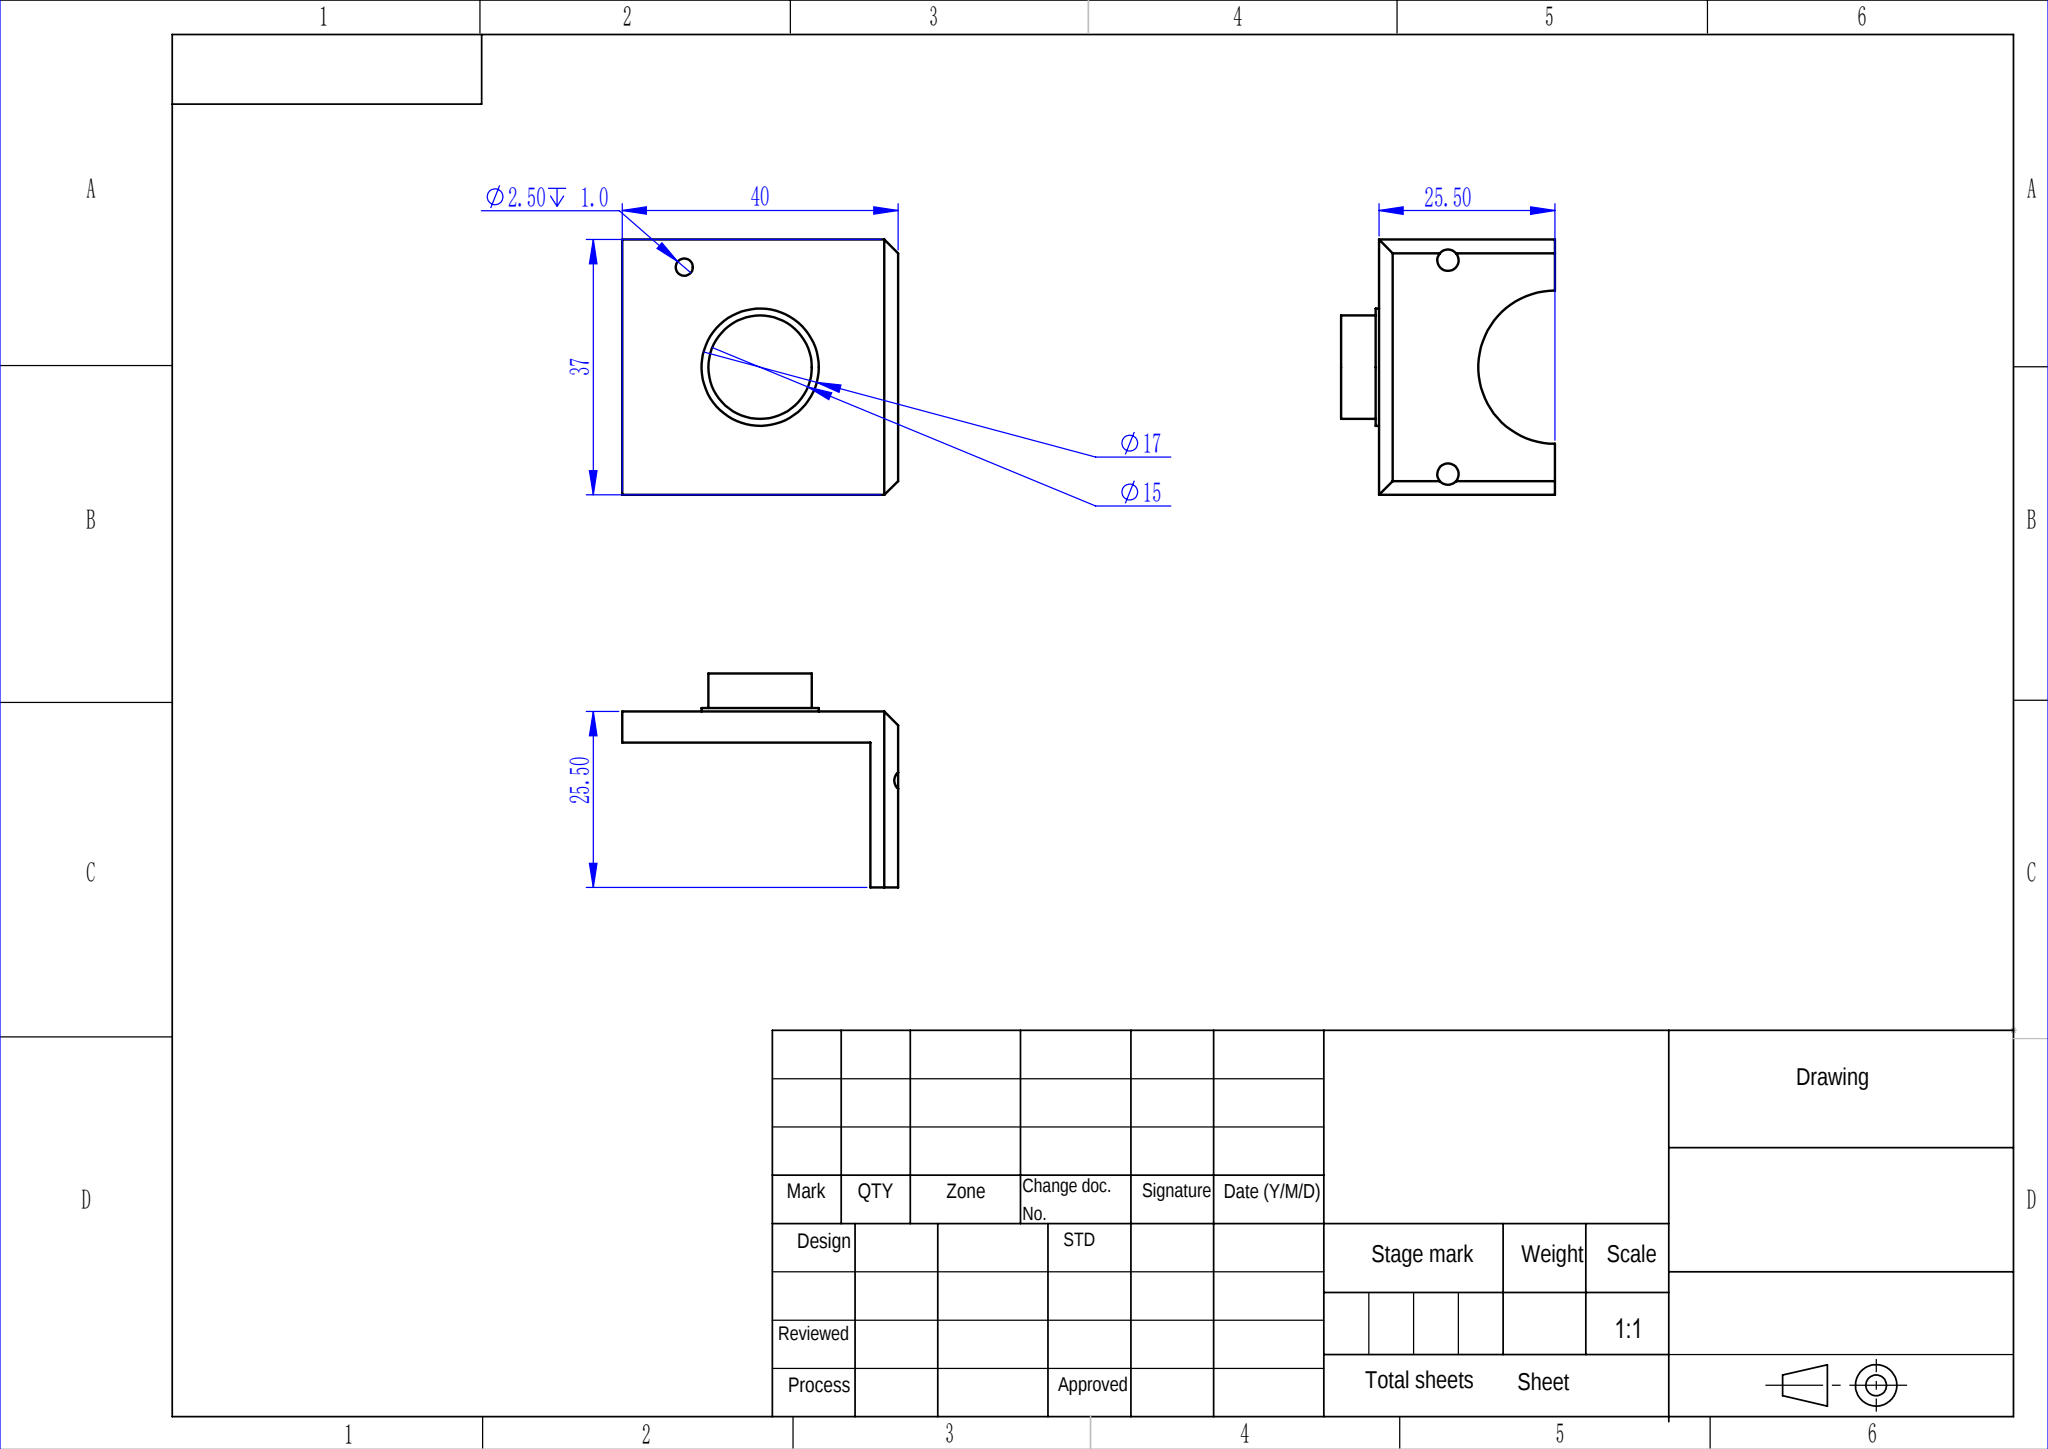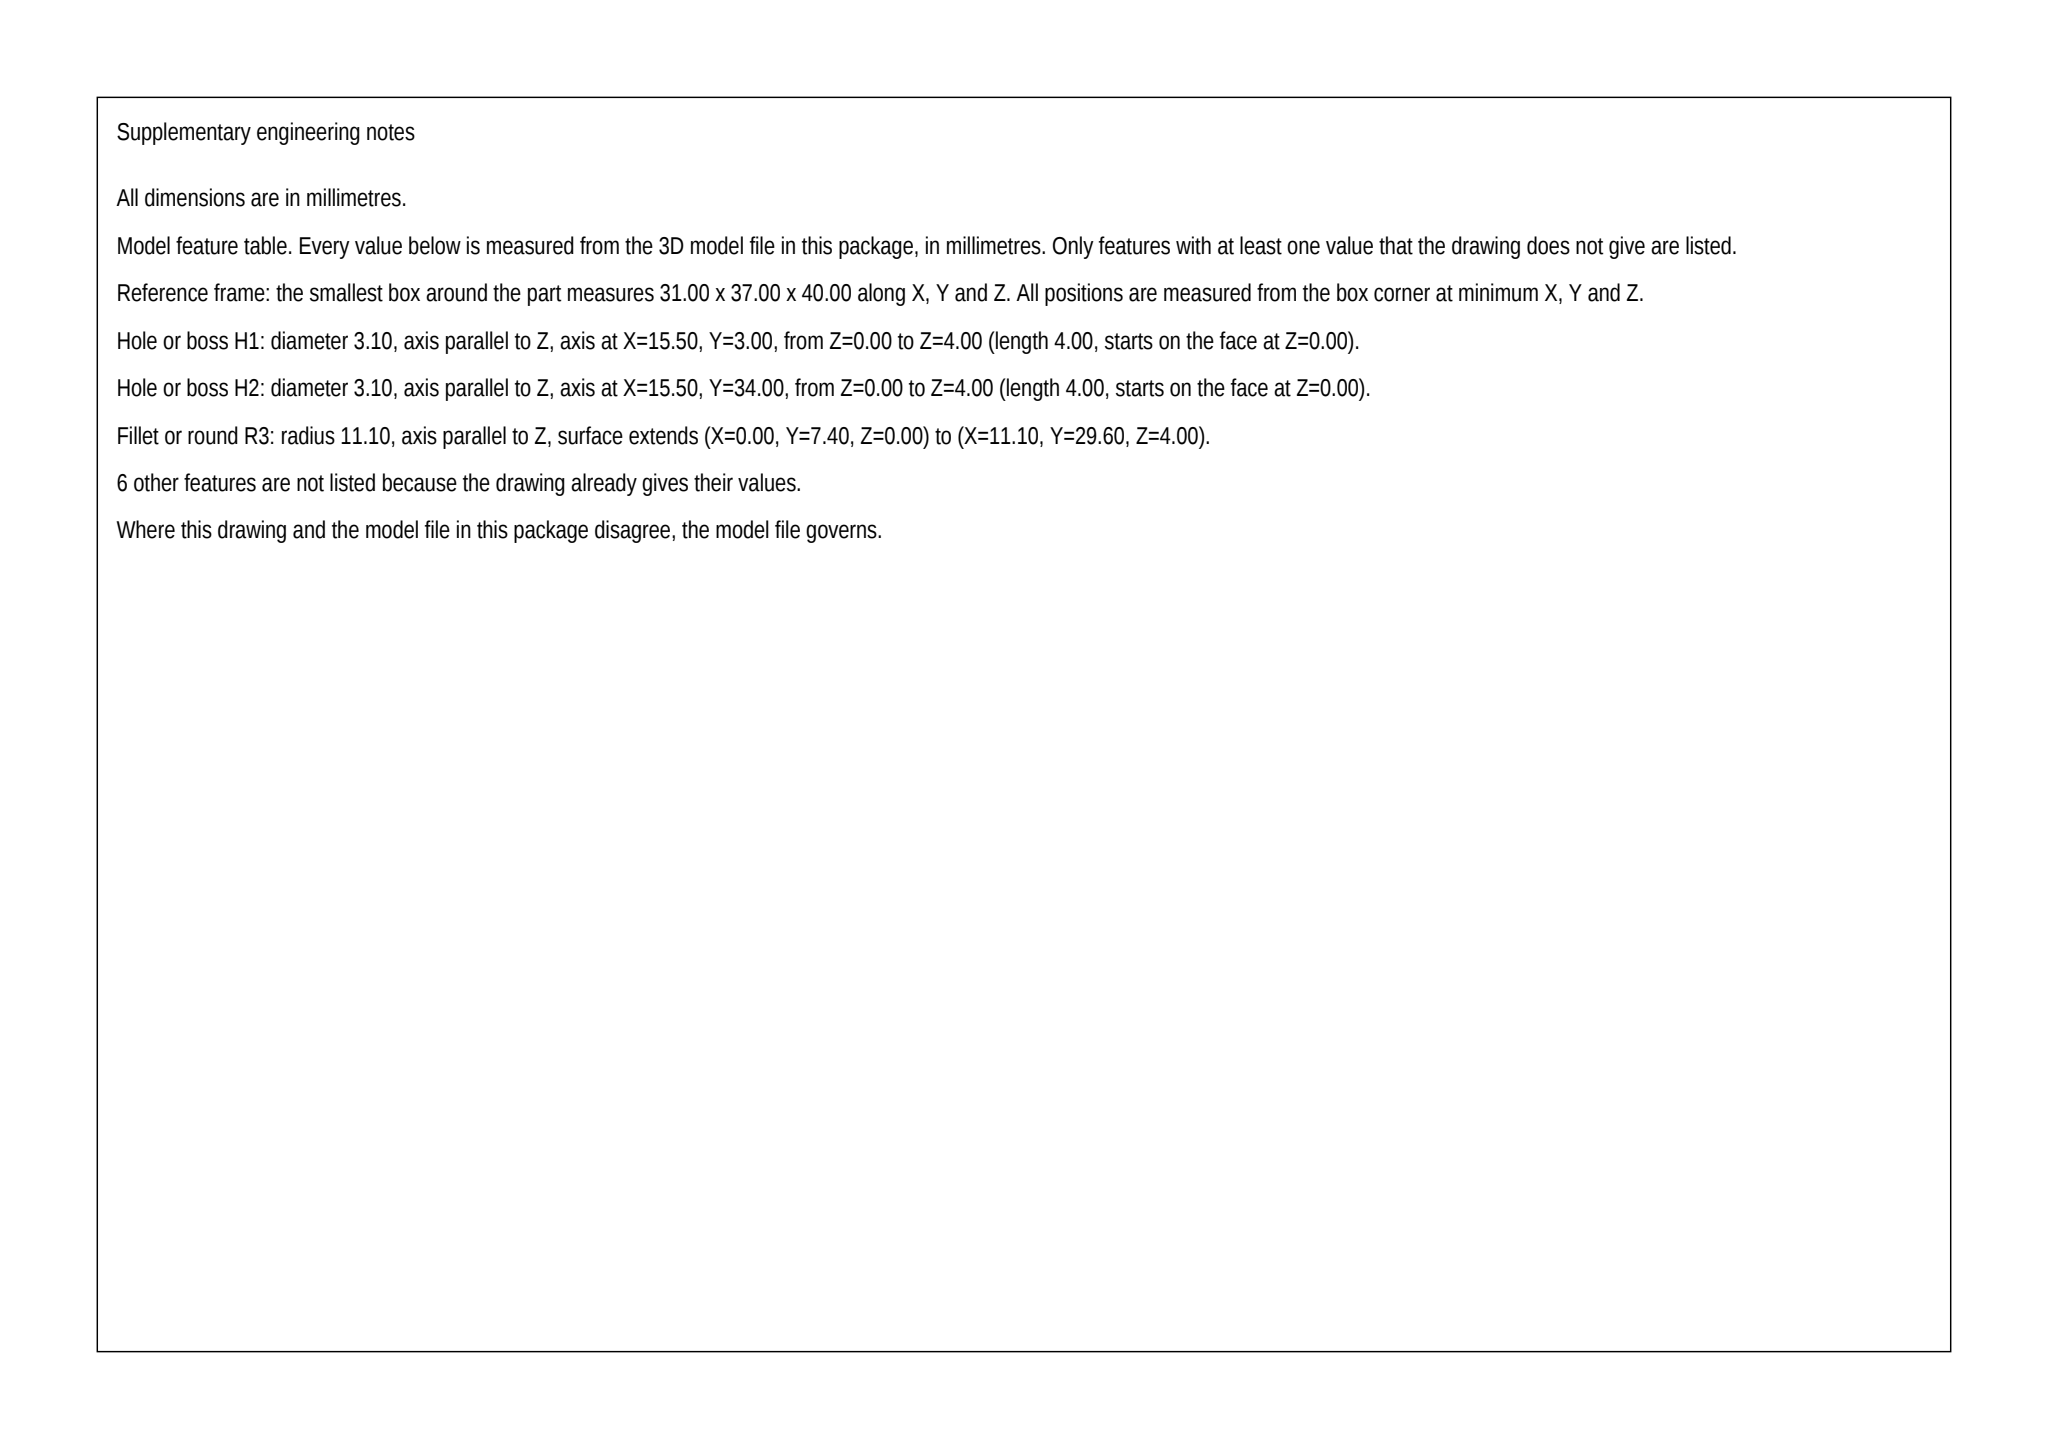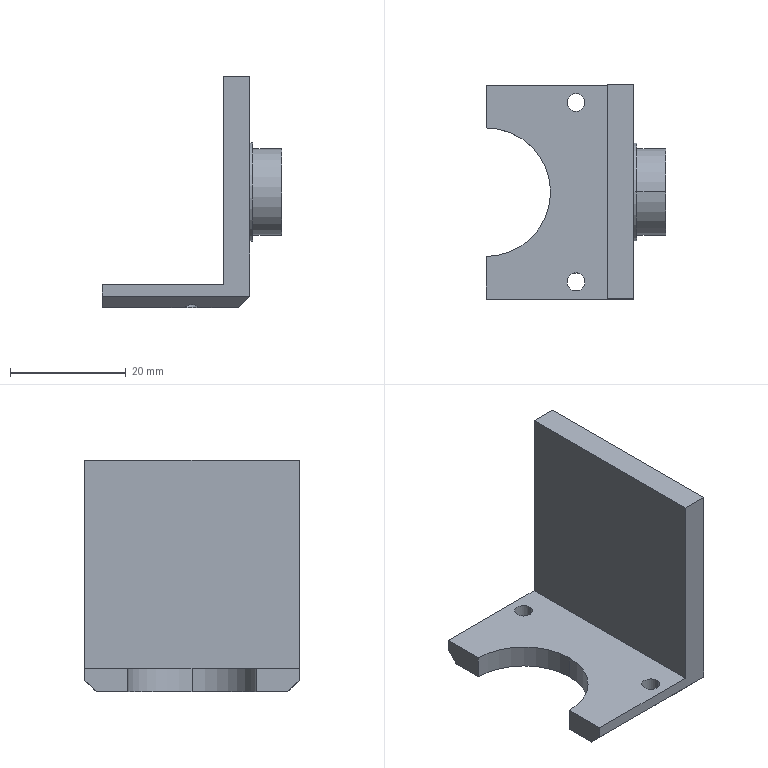Part | SolidWorks | mm | 1 solid | 27 faces | box 31 x 37 x 40 mm | volume 9755 mm3 | plane 15 | cylinder 12 | commonest cylinder face diameters 3.1 x4 2.5 x2 15 x2 17 x2 22.2 x2
STEP:
#1=CARTESIAN_POINT('',(3.5,33.,2.25));
#2=VERTEX_POINT('',#1);
#3=CARTESIAN_POINT('',(3.5,33.,-0.25));
#4=VERTEX_POINT('',#3);
#5=CARTESIAN_POINT('',(3.5,33.,1.));
#6=DIRECTION('',(1.,0.,0.));
#7=DIRECTION('',(0.,0.,-1.));
#8=AXIS2_PLACEMENT_3D('',#5,#6,#7);
#9=CIRCLE('',#8,1.25);
#10=EDGE_CURVE('',#2,#4,#9,.T.);
#11=ORIENTED_EDGE('',*,*,#10,.F.);
#12=CARTESIAN_POINT('',(4.5,33.,2.25));
#13=VERTEX_POINT('',#12);
#14=CARTESIAN_POINT('',(3.5,33.,2.25));
#15=DIRECTION('',(1.,0.,0.));
#16=VECTOR('',#15,1000.);
#17=LINE('',#14,#16);
#18=EDGE_CURVE('',#2,#13,#17,.T.);
#19=ORIENTED_EDGE('',*,*,#18,.T.);
#20=CARTESIAN_POINT('',(4.5,33.,-0.25));
#21=VERTEX_POINT('',#20);
#22=CARTESIAN_POINT('',(4.5,33.,1.));
#23=DIRECTION('',(1.,0.,0.));
#24=DIRECTION('',(0.,0.,-1.));
#25=AXIS2_PLACEMENT_3D('',#22,#23,#24);
#26=CIRCLE('',#25,1.25);
#27=EDGE_CURVE('',#13,#21,#26,.T.);
#28=ORIENTED_EDGE('',*,*,#27,.T.);
#29=CARTESIAN_POINT('',(3.5,33.,-0.25));
#30=DIRECTION('',(1.,0.,0.));
#31=VECTOR('',#30,1000.);
#32=LINE('',#29,#31);
#33=EDGE_CURVE('',#4,#21,#32,.T.);
#34=ORIENTED_EDGE('',*,*,#33,.F.);
#35=EDGE_LOOP('',(#11,#19,#28,#34));
#36=FACE_OUTER_BOUND('',#35,.T.);
#37=CARTESIAN_POINT('',(3.5,33.,1.));
#38=DIRECTION('',(1.,0.,0.));
#39=DIRECTION('',(0.,0.,-1.));
#40=AXIS2_PLACEMENT_3D('',#37,#38,#39);
#41=CYLINDRICAL_SURFACE('',#40,1.25);
#42=ADVANCED_FACE('',(#36),#41,.F.);
#43=CARTESIAN_POINT('',(10.,18.5,-17.5));
#44=VERTEX_POINT('',#43);
#45=CARTESIAN_POINT('',(10.,18.5,-2.5));
#46=VERTEX_POINT('',#45);
#47=CARTESIAN_POINT('',(10.,18.5,-10.));
#48=DIRECTION('',(1.,0.,0.));
#49=DIRECTION('',(0.,0.,-1.));
#50=AXIS2_PLACEMENT_3D('',#47,#48,#49);
#51=CIRCLE('',#50,7.5);
#52=EDGE_CURVE('',#44,#46,#51,.T.);
#53=ORIENTED_EDGE('',*,*,#52,.F.);
#54=CARTESIAN_POINT('',(5.,18.5,-17.5));
#55=VERTEX_POINT('',#54);
#56=CARTESIAN_POINT('',(10.,18.5,-17.5));
#57=DIRECTION('',(-1.,0.,0.));
#58=VECTOR('',#57,1000.);
#59=LINE('',#56,#58);
#60=EDGE_CURVE('',#44,#55,#59,.T.);
#61=ORIENTED_EDGE('',*,*,#60,.T.);
#62=CARTESIAN_POINT('',(5.,18.5,-2.5));
#63=VERTEX_POINT('',#62);
#64=CARTESIAN_POINT('',(5.,18.5,-10.));
#65=DIRECTION('',(1.,0.,0.));
#66=DIRECTION('',(0.,0.,-1.));
#67=AXIS2_PLACEMENT_3D('',#64,#65,#66);
#68=CIRCLE('',#67,7.5);
#69=EDGE_CURVE('',#55,#63,#68,.T.);
#70=ORIENTED_EDGE('',*,*,#69,.T.);
#71=CARTESIAN_POINT('',(10.,18.5,-2.5));
#72=DIRECTION('',(-1.,0.,0.));
#73=VECTOR('',#72,1000.);
#74=LINE('',#71,#73);
#75=EDGE_CURVE('',#46,#63,#74,.T.);
#76=ORIENTED_EDGE('',*,*,#75,.F.);
#77=EDGE_LOOP('',(#53,#61,#70,#76));
#78=FACE_OUTER_BOUND('',#77,.T.);
#79=CARTESIAN_POINT('',(10.,18.5,-10.));
#80=DIRECTION('',(-1.,0.,0.));
#81=DIRECTION('',(0.,0.,1.));
#82=AXIS2_PLACEMENT_3D('',#79,#80,#81);
#83=CYLINDRICAL_SURFACE('',#82,7.5);
#84=ADVANCED_FACE('',(#78),#83,.T.);
#85=CARTESIAN_POINT('',(5.,18.5,-18.5));
#86=VERTEX_POINT('',#85);
#87=CARTESIAN_POINT('',(5.,18.5,-1.5));
#88=VERTEX_POINT('',#87);
#89=CARTESIAN_POINT('',(5.,18.5,-10.));
#90=DIRECTION('',(1.,0.,0.));
#91=DIRECTION('',(0.,0.,-1.));
#92=AXIS2_PLACEMENT_3D('',#89,#90,#91);
#93=CIRCLE('',#92,8.5);
#94=EDGE_CURVE('',#86,#88,#93,.T.);
#95=ORIENTED_EDGE('',*,*,#94,.F.);
#96=CARTESIAN_POINT('',(4.5,18.5,-18.5));
#97=VERTEX_POINT('',#96);
#98=CARTESIAN_POINT('',(5.,18.5,-18.5));
#99=DIRECTION('',(-1.,0.,0.));
#100=VECTOR('',#99,1000.);
#101=LINE('',#98,#100);
#102=EDGE_CURVE('',#86,#97,#101,.T.);
#103=ORIENTED_EDGE('',*,*,#102,.T.);
#104=CARTESIAN_POINT('',(4.5,18.5,-1.5));
#105=VERTEX_POINT('',#104);
#106=CARTESIAN_POINT('',(4.5,18.5,-10.));
#107=DIRECTION('',(1.,0.,0.));
#108=DIRECTION('',(0.,0.,1.));
#109=AXIS2_PLACEMENT_3D('',#106,#107,#108);
#110=CIRCLE('',#109,8.5);
#111=EDGE_CURVE('',#97,#105,#110,.T.);
#112=ORIENTED_EDGE('',*,*,#111,.T.);
#113=CARTESIAN_POINT('',(5.,18.5,-1.5));
#114=DIRECTION('',(-1.,0.,0.));
#115=VECTOR('',#114,1000.);
#116=LINE('',#113,#115);
#117=EDGE_CURVE('',#88,#105,#116,.T.);
#118=ORIENTED_EDGE('',*,*,#117,.F.);
#119=EDGE_LOOP('',(#95,#103,#112,#118));
#120=FACE_OUTER_BOUND('',#119,.T.);
#121=CARTESIAN_POINT('',(5.,18.5,-10.));
#122=DIRECTION('',(-1.,0.,0.));
#123=DIRECTION('',(0.,0.,1.));
#124=AXIS2_PLACEMENT_3D('',#121,#122,#123);
#125=CYLINDRICAL_SURFACE('',#124,8.5);
#126=ADVANCED_FACE('',(#120),#125,.T.);
#127=CARTESIAN_POINT('',(-7.05,3.,-26.));
#128=VERTEX_POINT('',#127);
#129=CARTESIAN_POINT('',(-3.95,3.,-26.));
#130=VERTEX_POINT('',#129);
#131=CARTESIAN_POINT('',(-5.5,3.,-26.));
#132=DIRECTION('',(0.,0.,1.));
#133=DIRECTION('',(-1.,0.,0.));
#134=AXIS2_PLACEMENT_3D('',#131,#132,#133);
#135=CIRCLE('',#134,1.55);
#136=EDGE_CURVE('',#128,#130,#135,.T.);
#137=ORIENTED_EDGE('',*,*,#136,.T.);
#138=CARTESIAN_POINT('',(-3.95,3.,-30.));
#139=VERTEX_POINT('',#138);
#140=CARTESIAN_POINT('',(-3.95,3.,-21.616));
#141=DIRECTION('',(0.,0.,-1.));
#142=VECTOR('',#141,1000.);
#143=LINE('',#140,#142);
#144=EDGE_CURVE('',#130,#139,#143,.T.);
#145=ORIENTED_EDGE('',*,*,#144,.T.);
#146=CARTESIAN_POINT('',(-4.316,2.,-30.));
#147=VERTEX_POINT('',#146);
#148=CARTESIAN_POINT('',(-5.5,3.,-30.));
#149=DIRECTION('',(0.,0.,-1.));
#150=DIRECTION('',(-1.,0.,0.));
#151=AXIS2_PLACEMENT_3D('',#148,#149,#150);
#152=CIRCLE('',#151,1.55);
#153=EDGE_CURVE('',#139,#147,#152,.T.);
#154=ORIENTED_EDGE('',*,*,#153,.T.);
#155=CARTESIAN_POINT('',(-6.684,2.,-30.));
#156=VERTEX_POINT('',#155);
#157=CARTESIAN_POINT('',(-4.316,2.,-30.));
#158=CARTESIAN_POINT('',(-4.983,1.21,-29.21));
#159=CARTESIAN_POINT('',(-6.017,1.21,-29.21));
#160=CARTESIAN_POINT('',(-6.684,2.,-30.));
#161=(BOUNDED_CURVE()B_SPLINE_CURVE(3,(#157,#158,#159,#160),.UNSPECIFIED.,.F.,.T.)B_SPLINE_CURVE_WITH_KNOTS((4,4),(2.272,4.011),.UNSPECIFIED.)CURVE()GEOMETRIC_REPRESENTATION_ITEM()RATIONAL_B_SPLINE_CURVE((1.,0.7634,0.7634,1.))REPRESENTATION_ITEM(''));
#162=EDGE_CURVE('',#147,#156,#161,.T.);
#163=ORIENTED_EDGE('',*,*,#162,.T.);
#164=CARTESIAN_POINT('',(-7.05,3.,-30.));
#165=VERTEX_POINT('',#164);
#166=CARTESIAN_POINT('',(-5.5,3.,-30.));
#167=DIRECTION('',(0.,0.,-1.));
#168=DIRECTION('',(-1.,0.,0.));
#169=AXIS2_PLACEMENT_3D('',#166,#167,#168);
#170=CIRCLE('',#169,1.55);
#171=EDGE_CURVE('',#156,#165,#170,.T.);
#172=ORIENTED_EDGE('',*,*,#171,.T.);
#173=CARTESIAN_POINT('',(-7.05,3.,-21.616));
#174=DIRECTION('',(0.,0.,-1.));
#175=VECTOR('',#174,1000.);
#176=LINE('',#173,#175);
#177=EDGE_CURVE('',#128,#165,#176,.T.);
#178=ORIENTED_EDGE('',*,*,#177,.F.);
#179=EDGE_LOOP('',(#137,#145,#154,#163,#172,#178));
#180=FACE_OUTER_BOUND('',#179,.T.);
#181=CARTESIAN_POINT('',(-5.5,3.,-21.616));
#182=DIRECTION('',(0.,0.,-1.));
#183=DIRECTION('',(-1.,0.,0.));
#184=AXIS2_PLACEMENT_3D('',#181,#182,#183);
#185=CYLINDRICAL_SURFACE('',#184,1.55);
#186=ADVANCED_FACE('',(#180),#185,.F.);
#187=CARTESIAN_POINT('',(-7.05,34.,-26.));
#188=VERTEX_POINT('',#187);
#189=CARTESIAN_POINT('',(-3.95,34.,-26.));
#190=VERTEX_POINT('',#189);
#191=CARTESIAN_POINT('',(-5.5,34.,-26.));
#192=DIRECTION('',(0.,0.,1.));
#193=DIRECTION('',(-1.,0.,0.));
#194=AXIS2_PLACEMENT_3D('',#191,#192,#193);
#195=CIRCLE('',#194,1.55);
#196=EDGE_CURVE('',#188,#190,#195,.T.);
#197=ORIENTED_EDGE('',*,*,#196,.T.);
#198=CARTESIAN_POINT('',(-3.95,34.,-30.));
#199=VERTEX_POINT('',#198);
#200=CARTESIAN_POINT('',(-3.95,34.,-21.616));
#201=DIRECTION('',(0.,0.,-1.));
#202=VECTOR('',#201,1000.);
#203=LINE('',#200,#202);
#204=EDGE_CURVE('',#190,#199,#203,.T.);
#205=ORIENTED_EDGE('',*,*,#204,.T.);
#206=CARTESIAN_POINT('',(-7.05,34.,-30.));
#207=VERTEX_POINT('',#206);
#208=CARTESIAN_POINT('',(-5.5,34.,-30.));
#209=DIRECTION('',(0.,0.,-1.));
#210=DIRECTION('',(-1.,0.,0.));
#211=AXIS2_PLACEMENT_3D('',#208,#209,#210);
#212=CIRCLE('',#211,1.55);
#213=EDGE_CURVE('',#199,#207,#212,.T.);
#214=ORIENTED_EDGE('',*,*,#213,.T.);
#215=CARTESIAN_POINT('',(-7.05,34.,-21.616));
#216=DIRECTION('',(0.,0.,-1.));
#217=VECTOR('',#216,1000.);
#218=LINE('',#215,#217);
#219=EDGE_CURVE('',#188,#207,#218,.T.);
#220=ORIENTED_EDGE('',*,*,#219,.F.);
#221=EDGE_LOOP('',(#197,#205,#214,#220));
#222=FACE_OUTER_BOUND('',#221,.T.);
#223=CARTESIAN_POINT('',(-5.5,34.,-21.616));
#224=DIRECTION('',(0.,0.,-1.));
#225=DIRECTION('',(-1.,0.,0.));
#226=AXIS2_PLACEMENT_3D('',#223,#224,#225);
#227=CYLINDRICAL_SURFACE('',#226,1.55);
#228=ADVANCED_FACE('',(#222),#227,.F.);
#229=CARTESIAN_POINT('',(-21.,29.6,-30.));
#230=VERTEX_POINT('',#229);
#231=CARTESIAN_POINT('',(-9.9,18.5,-30.));
#232=VERTEX_POINT('',#231);
#233=CARTESIAN_POINT('',(-21.,18.5,-30.));
#234=DIRECTION('',(0.,0.,-1.));
#235=DIRECTION('',(1.,0.,0.));
#236=AXIS2_PLACEMENT_3D('',#233,#234,#235);
#237=CIRCLE('',#236,11.1);
#238=EDGE_CURVE('',#230,#232,#237,.T.);
#239=ORIENTED_EDGE('',*,*,#238,.T.);
#240=CARTESIAN_POINT('',(-9.9,18.5,-26.));
#241=VERTEX_POINT('',#240);
#242=CARTESIAN_POINT('',(-9.9,18.5,-61.396));
#243=DIRECTION('',(0.,0.,1.));
#244=VECTOR('',#243,1000.);
#245=LINE('',#242,#244);
#246=EDGE_CURVE('',#232,#241,#245,.T.);
#247=ORIENTED_EDGE('',*,*,#246,.T.);
#248=CARTESIAN_POINT('',(-21.,29.6,-26.));
#249=VERTEX_POINT('',#248);
#250=CARTESIAN_POINT('',(-21.,18.5,-26.));
#251=DIRECTION('',(0.,0.,1.));
#252=DIRECTION('',(1.,0.,0.));
#253=AXIS2_PLACEMENT_3D('',#250,#251,#252);
#254=CIRCLE('',#253,11.1);
#255=EDGE_CURVE('',#241,#249,#254,.T.);
#256=ORIENTED_EDGE('',*,*,#255,.T.);
#257=CARTESIAN_POINT('',(-21.,29.6,-61.396));
#258=DIRECTION('',(0.,0.,1.));
#259=VECTOR('',#258,1000.);
#260=LINE('',#257,#259);
#261=EDGE_CURVE('',#230,#249,#260,.T.);
#262=ORIENTED_EDGE('',*,*,#261,.F.);
#263=EDGE_LOOP('',(#239,#247,#256,#262));
#264=FACE_OUTER_BOUND('',#263,.T.);
#265=CARTESIAN_POINT('',(-21.,18.5,-61.396));
#266=DIRECTION('',(0.,0.,1.));
#267=DIRECTION('',(1.,0.,0.));
#268=AXIS2_PLACEMENT_3D('',#265,#266,#267);
#269=CYLINDRICAL_SURFACE('',#268,11.1);
#270=ADVANCED_FACE('',(#264),#269,.F.);
#271=CARTESIAN_POINT('',(-21.,0.,-28.));
#272=VERTEX_POINT('',#271);
#273=CARTESIAN_POINT('',(-21.,0.,-26.));
#274=VERTEX_POINT('',#273);
#275=CARTESIAN_POINT('',(-21.,0.,0.));
#276=DIRECTION('',(0.,0.,1.));
#277=VECTOR('',#276,1000.);
#278=LINE('',#275,#277);
#279=EDGE_CURVE('',#272,#274,#278,.T.);
#280=ORIENTED_EDGE('',*,*,#279,.F.);
#281=CARTESIAN_POINT('',(4.5,0.,-28.));
#282=VERTEX_POINT('',#281);
#283=CARTESIAN_POINT('',(4.5,0.,-28.));
#284=DIRECTION('',(1.,0.,0.));
#285=VECTOR('',#284,1000.);
#286=LINE('',#283,#285);
#287=EDGE_CURVE('',#272,#282,#286,.T.);
#288=ORIENTED_EDGE('',*,*,#287,.T.);
#289=CARTESIAN_POINT('',(4.5,0.,10.));
#290=VERTEX_POINT('',#289);
#291=CARTESIAN_POINT('',(4.5,0.,0.));
#292=DIRECTION('',(0.,0.,-1.));
#293=VECTOR('',#292,1000.);
#294=LINE('',#291,#293);
#295=EDGE_CURVE('',#290,#282,#294,.T.);
#296=ORIENTED_EDGE('',*,*,#295,.F.);
#297=CARTESIAN_POINT('',(0.,0.,10.));
#298=VERTEX_POINT('',#297);
#299=CARTESIAN_POINT('',(4.5,0.,10.));
#300=DIRECTION('',(1.,0.,0.));
#301=VECTOR('',#300,1000.);
#302=LINE('',#299,#301);
#303=EDGE_CURVE('',#298,#290,#302,.T.);
#304=ORIENTED_EDGE('',*,*,#303,.F.);
#305=CARTESIAN_POINT('',(0.,0.,-26.));
#306=VERTEX_POINT('',#305);
#307=CARTESIAN_POINT('',(0.,0.,0.));
#308=DIRECTION('',(0.,0.,-1.));
#309=VECTOR('',#308,1000.);
#310=LINE('',#307,#309);
#311=EDGE_CURVE('',#298,#306,#310,.T.);
#312=ORIENTED_EDGE('',*,*,#311,.T.);
#313=CARTESIAN_POINT('',(-42.,0.,-26.));
#314=DIRECTION('',(1.,0.,0.));
#315=VECTOR('',#314,1000.);
#316=LINE('',#313,#315);
#317=EDGE_CURVE('',#274,#306,#316,.T.);
#318=ORIENTED_EDGE('',*,*,#317,.F.);
#319=EDGE_LOOP('',(#280,#288,#296,#304,#312,#318));
#320=FACE_OUTER_BOUND('',#319,.T.);
#321=CARTESIAN_POINT('',(4.5,0.,0.));
#322=DIRECTION('',(0.,1.,0.));
#323=DIRECTION('',(0.,0.,1.));
#324=AXIS2_PLACEMENT_3D('',#321,#322,#323);
#325=PLANE('',#324);
#326=ADVANCED_FACE('',(#320),#325,.F.);
#327=CARTESIAN_POINT('',(-21.,35.,-30.));
#328=VERTEX_POINT('',#327);
#329=CARTESIAN_POINT('',(-21.,0.,-30.));
#330=DIRECTION('',(0.,-1.,0.));
#331=VECTOR('',#330,1000.);
#332=LINE('',#329,#331);
#333=EDGE_CURVE('',#328,#230,#332,.T.);
#334=ORIENTED_EDGE('',*,*,#333,.F.);
#335=CARTESIAN_POINT('',(-6.684,35.,-30.));
#336=VERTEX_POINT('',#335);
#337=CARTESIAN_POINT('',(4.5,35.,-30.));
#338=DIRECTION('',(1.,0.,0.));
#339=VECTOR('',#338,1000.);
#340=LINE('',#337,#339);
#341=EDGE_CURVE('',#328,#336,#340,.T.);
#342=ORIENTED_EDGE('',*,*,#341,.T.);
#343=CARTESIAN_POINT('',(-5.5,34.,-30.));
#344=DIRECTION('',(0.,0.,-1.));
#345=DIRECTION('',(-1.,0.,0.));
#346=AXIS2_PLACEMENT_3D('',#343,#344,#345);
#347=CIRCLE('',#346,1.55);
#348=EDGE_CURVE('',#207,#336,#347,.T.);
#349=ORIENTED_EDGE('',*,*,#348,.F.);
#350=ORIENTED_EDGE('',*,*,#213,.F.);
#351=CARTESIAN_POINT('',(-4.316,35.,-30.));
#352=VERTEX_POINT('',#351);
#353=CARTESIAN_POINT('',(-5.5,34.,-30.));
#354=DIRECTION('',(0.,0.,-1.));
#355=DIRECTION('',(-1.,0.,0.));
#356=AXIS2_PLACEMENT_3D('',#353,#354,#355);
#357=CIRCLE('',#356,1.55);
#358=EDGE_CURVE('',#352,#199,#357,.T.);
#359=ORIENTED_EDGE('',*,*,#358,.F.);
#360=CARTESIAN_POINT('',(2.5,35.,-30.));
#361=VERTEX_POINT('',#360);
#362=CARTESIAN_POINT('',(4.5,35.,-30.));
#363=DIRECTION('',(1.,0.,0.));
#364=VECTOR('',#363,1000.);
#365=LINE('',#362,#364);
#366=EDGE_CURVE('',#352,#361,#365,.T.);
#367=ORIENTED_EDGE('',*,*,#366,.T.);
#368=CARTESIAN_POINT('',(2.5,2.,-30.));
#369=VERTEX_POINT('',#368);
#370=CARTESIAN_POINT('',(2.5,0.,-30.));
#371=DIRECTION('',(0.,-1.,0.));
#372=VECTOR('',#371,1000.);
#373=LINE('',#370,#372);
#374=EDGE_CURVE('',#361,#369,#373,.T.);
#375=ORIENTED_EDGE('',*,*,#374,.T.);
#376=CARTESIAN_POINT('',(4.5,2.,-30.));
#377=DIRECTION('',(-1.,0.,0.));
#378=VECTOR('',#377,1000.);
#379=LINE('',#376,#378);
#380=EDGE_CURVE('',#369,#147,#379,.T.);
#381=ORIENTED_EDGE('',*,*,#380,.T.);
#382=ORIENTED_EDGE('',*,*,#153,.F.);
#383=CARTESIAN_POINT('',(-5.5,3.,-30.));
#384=DIRECTION('',(0.,0.,-1.));
#385=DIRECTION('',(-1.,0.,0.));
#386=AXIS2_PLACEMENT_3D('',#383,#384,#385);
#387=CIRCLE('',#386,1.55);
#388=EDGE_CURVE('',#165,#139,#387,.T.);
#389=ORIENTED_EDGE('',*,*,#388,.F.);
#390=ORIENTED_EDGE('',*,*,#171,.F.);
#391=CARTESIAN_POINT('',(-21.,2.,-30.));
#392=VERTEX_POINT('',#391);
#393=CARTESIAN_POINT('',(4.5,2.,-30.));
#394=DIRECTION('',(-1.,0.,0.));
#395=VECTOR('',#394,1000.);
#396=LINE('',#393,#395);
#397=EDGE_CURVE('',#156,#392,#396,.T.);
#398=ORIENTED_EDGE('',*,*,#397,.T.);
#399=CARTESIAN_POINT('',(-21.,7.4,-30.));
#400=VERTEX_POINT('',#399);
#401=CARTESIAN_POINT('',(-21.,0.,-30.));
#402=DIRECTION('',(0.,-1.,0.));
#403=VECTOR('',#402,1000.);
#404=LINE('',#401,#403);
#405=EDGE_CURVE('',#400,#392,#404,.T.);
#406=ORIENTED_EDGE('',*,*,#405,.F.);
#407=CARTESIAN_POINT('',(-21.,18.5,-30.));
#408=DIRECTION('',(0.,0.,-1.));
#409=DIRECTION('',(1.,0.,0.));
#410=AXIS2_PLACEMENT_3D('',#407,#408,#409);
#411=CIRCLE('',#410,11.1);
#412=EDGE_CURVE('',#232,#400,#411,.T.);
#413=ORIENTED_EDGE('',*,*,#412,.F.);
#414=ORIENTED_EDGE('',*,*,#238,.F.);
#415=EDGE_LOOP('',(#334,#342,#349,#350,#359,#367,#375,#381,#382,#389,#390,#398,#406,#413,#414));
#416=FACE_OUTER_BOUND('',#415,.T.);
#417=CARTESIAN_POINT('',(4.5,0.,-30.));
#418=DIRECTION('',(0.,0.,1.));
#419=DIRECTION('',(1.,0.,0.));
#420=AXIS2_PLACEMENT_3D('',#417,#418,#419);
#421=PLANE('',#420);
#422=ADVANCED_FACE('',(#416),#421,.F.);
#423=CARTESIAN_POINT('',(-21.,37.,-26.));
#424=VERTEX_POINT('',#423);
#425=CARTESIAN_POINT('',(-21.,37.,-28.));
#426=VERTEX_POINT('',#425);
#427=CARTESIAN_POINT('',(-21.,37.,0.));
#428=DIRECTION('',(0.,0.,-1.));
#429=VECTOR('',#428,1000.);
#430=LINE('',#427,#429);
#431=EDGE_CURVE('',#424,#426,#430,.T.);
#432=ORIENTED_EDGE('',*,*,#431,.F.);
#433=CARTESIAN_POINT('',(0.,37.,-26.));
#434=VERTEX_POINT('',#433);
#435=CARTESIAN_POINT('',(-42.,37.,-26.));
#436=DIRECTION('',(1.,0.,0.));
#437=VECTOR('',#436,1000.);
#438=LINE('',#435,#437);
#439=EDGE_CURVE('',#424,#434,#438,.T.);
#440=ORIENTED_EDGE('',*,*,#439,.T.);
#441=CARTESIAN_POINT('',(0.,37.,10.));
#442=VERTEX_POINT('',#441);
#443=CARTESIAN_POINT('',(0.,37.,0.));
#444=DIRECTION('',(0.,0.,1.));
#445=VECTOR('',#444,1000.);
#446=LINE('',#443,#445);
#447=EDGE_CURVE('',#434,#442,#446,.T.);
#448=ORIENTED_EDGE('',*,*,#447,.T.);
#449=CARTESIAN_POINT('',(4.5,37.,10.));
#450=VERTEX_POINT('',#449);
#451=CARTESIAN_POINT('',(0.,37.,10.));
#452=DIRECTION('',(-1.,0.,0.));
#453=VECTOR('',#452,1000.);
#454=LINE('',#451,#453);
#455=EDGE_CURVE('',#450,#442,#454,.T.);
#456=ORIENTED_EDGE('',*,*,#455,.F.);
#457=CARTESIAN_POINT('',(4.5,37.,-28.));
#458=VERTEX_POINT('',#457);
#459=CARTESIAN_POINT('',(4.5,37.,0.));
#460=DIRECTION('',(0.,0.,1.));
#461=VECTOR('',#460,1000.);
#462=LINE('',#459,#461);
#463=EDGE_CURVE('',#458,#450,#462,.T.);
#464=ORIENTED_EDGE('',*,*,#463,.F.);
#465=CARTESIAN_POINT('',(4.5,37.,-28.));
#466=DIRECTION('',(-1.,0.,0.));
#467=VECTOR('',#466,1000.);
#468=LINE('',#465,#467);
#469=EDGE_CURVE('',#458,#426,#468,.T.);
#470=ORIENTED_EDGE('',*,*,#469,.T.);
#471=EDGE_LOOP('',(#432,#440,#448,#456,#464,#470));
#472=FACE_OUTER_BOUND('',#471,.T.);
#473=CARTESIAN_POINT('',(4.5,37.,0.));
#474=DIRECTION('',(0.,-1.,0.));
#475=DIRECTION('',(0.,0.,-1.));
#476=AXIS2_PLACEMENT_3D('',#473,#474,#475);
#477=PLANE('',#476);
#478=ADVANCED_FACE('',(#472),#477,.F.);
#479=ORIENTED_EDGE('',*,*,#196,.F.);
#480=CARTESIAN_POINT('',(-5.5,34.,-26.));
#481=DIRECTION('',(0.,0.,1.));
#482=DIRECTION('',(-1.,0.,0.));
#483=AXIS2_PLACEMENT_3D('',#480,#481,#482);
#484=CIRCLE('',#483,1.55);
#485=EDGE_CURVE('',#190,#188,#484,.T.);
#486=ORIENTED_EDGE('',*,*,#485,.F.);
#487=EDGE_LOOP('',(#479,#486));
#488=FACE_BOUND('',#487,.T.);
#489=ORIENTED_EDGE('',*,*,#136,.F.);
#490=CARTESIAN_POINT('',(-5.5,3.,-26.));
#491=DIRECTION('',(0.,0.,1.));
#492=DIRECTION('',(-1.,0.,0.));
#493=AXIS2_PLACEMENT_3D('',#490,#491,#492);
#494=CIRCLE('',#493,1.55);
#495=EDGE_CURVE('',#130,#128,#494,.T.);
#496=ORIENTED_EDGE('',*,*,#495,.F.);
#497=EDGE_LOOP('',(#489,#496));
#498=FACE_BOUND('',#497,.T.);
#499=CARTESIAN_POINT('',(-21.,7.4,-26.));
#500=VERTEX_POINT('',#499);
#501=CARTESIAN_POINT('',(-21.,37.,-26.));
#502=DIRECTION('',(0.,1.,0.));
#503=VECTOR('',#502,1000.);
#504=LINE('',#501,#503);
#505=EDGE_CURVE('',#274,#500,#504,.T.);
#506=ORIENTED_EDGE('',*,*,#505,.F.);
#507=ORIENTED_EDGE('',*,*,#317,.T.);
#508=CARTESIAN_POINT('',(0.,37.,-26.));
#509=DIRECTION('',(0.,1.,0.));
#510=VECTOR('',#509,1000.);
#511=LINE('',#508,#510);
#512=EDGE_CURVE('',#306,#434,#511,.T.);
#513=ORIENTED_EDGE('',*,*,#512,.T.);
#514=ORIENTED_EDGE('',*,*,#439,.F.);
#515=CARTESIAN_POINT('',(-21.,37.,-26.));
#516=DIRECTION('',(0.,1.,0.));
#517=VECTOR('',#516,1000.);
#518=LINE('',#515,#517);
#519=EDGE_CURVE('',#249,#424,#518,.T.);
#520=ORIENTED_EDGE('',*,*,#519,.F.);
#521=ORIENTED_EDGE('',*,*,#255,.F.);
#522=CARTESIAN_POINT('',(-21.,18.5,-26.));
#523=DIRECTION('',(0.,0.,1.));
#524=DIRECTION('',(1.,0.,0.));
#525=AXIS2_PLACEMENT_3D('',#522,#523,#524);
#526=CIRCLE('',#525,11.1);
#527=EDGE_CURVE('',#500,#241,#526,.T.);
#528=ORIENTED_EDGE('',*,*,#527,.F.);
#529=EDGE_LOOP('',(#506,#507,#513,#514,#520,#521,#528));
#530=FACE_OUTER_BOUND('',#529,.T.);
#531=CARTESIAN_POINT('',(-42.,37.,-26.));
#532=DIRECTION('',(0.,0.,-1.));
#533=DIRECTION('',(-1.,0.,0.));
#534=AXIS2_PLACEMENT_3D('',#531,#532,#533);
#535=PLANE('',#534);
#536=ADVANCED_FACE('',(#488,#498,#530),#535,.F.);
#537=ORIENTED_EDGE('',*,*,#246,.F.);
#538=ORIENTED_EDGE('',*,*,#412,.T.);
#539=CARTESIAN_POINT('',(-21.,7.4,-61.396));
#540=DIRECTION('',(0.,0.,-1.));
#541=VECTOR('',#540,1000.);
#542=LINE('',#539,#541);
#543=EDGE_CURVE('',#500,#400,#542,.T.);
#544=ORIENTED_EDGE('',*,*,#543,.F.);
#545=ORIENTED_EDGE('',*,*,#527,.T.);
#546=EDGE_LOOP('',(#537,#538,#544,#545));
#547=FACE_OUTER_BOUND('',#546,.T.);
#548=CARTESIAN_POINT('',(-21.,18.5,-61.396));
#549=DIRECTION('',(0.,0.,1.));
#550=DIRECTION('',(1.,0.,0.));
#551=AXIS2_PLACEMENT_3D('',#548,#549,#550);
#552=CYLINDRICAL_SURFACE('',#551,11.1);
#553=ADVANCED_FACE('',(#547),#552,.F.);
#554=ORIENTED_EDGE('',*,*,#341,.F.);
#555=CARTESIAN_POINT('',(-21.,37.,-28.));
#556=DIRECTION('',(0.,0.7071,0.7071));
#557=VECTOR('',#556,1000.);
#558=LINE('',#555,#557);
#559=EDGE_CURVE('',#328,#426,#558,.T.);
#560=ORIENTED_EDGE('',*,*,#559,.T.);
#561=ORIENTED_EDGE('',*,*,#469,.F.);
#562=CARTESIAN_POINT('',(4.5,37.,-28.));
#563=DIRECTION('',(0.5774,0.5774,0.5774));
#564=VECTOR('',#563,1000.);
#565=LINE('',#562,#564);
#566=EDGE_CURVE('',#361,#458,#565,.T.);
#567=ORIENTED_EDGE('',*,*,#566,.F.);
#568=ORIENTED_EDGE('',*,*,#366,.F.);
#569=CARTESIAN_POINT('',(-6.684,35.,-30.));
#570=CARTESIAN_POINT('',(-6.017,35.79,-29.21));
#571=CARTESIAN_POINT('',(-4.983,35.79,-29.21));
#572=CARTESIAN_POINT('',(-4.316,35.,-30.));
#573=(BOUNDED_CURVE()B_SPLINE_CURVE(3,(#569,#570,#571,#572),.UNSPECIFIED.,.F.,.T.)B_SPLINE_CURVE_WITH_KNOTS((4,4),(2.272,4.011),.UNSPECIFIED.)CURVE()GEOMETRIC_REPRESENTATION_ITEM()RATIONAL_B_SPLINE_CURVE((1.,0.7634,0.7634,1.))REPRESENTATION_ITEM(''));
#574=EDGE_CURVE('',#336,#352,#573,.T.);
#575=ORIENTED_EDGE('',*,*,#574,.F.);
#576=EDGE_LOOP('',(#554,#560,#561,#567,#568,#575));
#577=FACE_OUTER_BOUND('',#576,.T.);
#578=CARTESIAN_POINT('',(4.5,37.,-28.));
#579=DIRECTION('',(0.,-0.7071,0.7071));
#580=DIRECTION('',(-1.,0.,0.));
#581=AXIS2_PLACEMENT_3D('',#578,#579,#580);
#582=PLANE('',#581);
#583=ADVANCED_FACE('',(#577),#582,.F.);
#584=ORIENTED_EDGE('',*,*,#287,.F.);
#585=CARTESIAN_POINT('',(-21.,2.,-30.));
#586=DIRECTION('',(0.,0.7071,-0.7071));
#587=VECTOR('',#586,1000.);
#588=LINE('',#585,#587);
#589=EDGE_CURVE('',#272,#392,#588,.T.);
#590=ORIENTED_EDGE('',*,*,#589,.T.);
#591=ORIENTED_EDGE('',*,*,#397,.F.);
#592=ORIENTED_EDGE('',*,*,#162,.F.);
#593=ORIENTED_EDGE('',*,*,#380,.F.);
#594=CARTESIAN_POINT('',(4.5,-0.,-28.));
#595=DIRECTION('',(0.5774,-0.5774,0.5774));
#596=VECTOR('',#595,1000.);
#597=LINE('',#594,#596);
#598=EDGE_CURVE('',#369,#282,#597,.T.);
#599=ORIENTED_EDGE('',*,*,#598,.T.);
#600=EDGE_LOOP('',(#584,#590,#591,#592,#593,#599));
#601=FACE_OUTER_BOUND('',#600,.T.);
#602=CARTESIAN_POINT('',(4.5,2.,-30.));
#603=DIRECTION('',(0.,0.7071,0.7071));
#604=DIRECTION('',(-1.,0.,0.));
#605=AXIS2_PLACEMENT_3D('',#602,#603,#604);
#606=PLANE('',#605);
#607=ADVANCED_FACE('',(#601),#606,.F.);
#608=CARTESIAN_POINT('',(4.5,33.,1.));
#609=DIRECTION('',(1.,0.,0.));
#610=DIRECTION('',(0.,0.,-1.));
#611=AXIS2_PLACEMENT_3D('',#608,#609,#610);
#612=CIRCLE('',#611,1.25);
#613=EDGE_CURVE('',#21,#13,#612,.T.);
#614=ORIENTED_EDGE('',*,*,#613,.F.);
#615=ORIENTED_EDGE('',*,*,#27,.F.);
#616=EDGE_LOOP('',(#614,#615));
#617=FACE_BOUND('',#616,.T.);
#618=CARTESIAN_POINT('',(4.5,18.5,-10.));
#619=DIRECTION('',(1.,0.,0.));
#620=DIRECTION('',(0.,0.,1.));
#621=AXIS2_PLACEMENT_3D('',#618,#619,#620);
#622=CIRCLE('',#621,8.5);
#623=EDGE_CURVE('',#105,#97,#622,.T.);
#624=ORIENTED_EDGE('',*,*,#623,.F.);
#625=ORIENTED_EDGE('',*,*,#111,.F.);
#626=EDGE_LOOP('',(#624,#625));
#627=FACE_BOUND('',#626,.T.);
#628=ORIENTED_EDGE('',*,*,#295,.T.);
#629=CARTESIAN_POINT('',(4.5,0.,-28.));
#630=DIRECTION('',(0.,1.,0.));
#631=VECTOR('',#630,1000.);
#632=LINE('',#629,#631);
#633=EDGE_CURVE('',#282,#458,#632,.T.);
#634=ORIENTED_EDGE('',*,*,#633,.T.);
#635=ORIENTED_EDGE('',*,*,#463,.T.);
#636=CARTESIAN_POINT('',(4.5,37.,10.));
#637=DIRECTION('',(0.,1.,0.));
#638=VECTOR('',#637,1000.);
#639=LINE('',#636,#638);
#640=EDGE_CURVE('',#290,#450,#639,.T.);
#641=ORIENTED_EDGE('',*,*,#640,.F.);
#642=EDGE_LOOP('',(#628,#634,#635,#641));
#643=FACE_OUTER_BOUND('',#642,.T.);
#644=CARTESIAN_POINT('',(4.5,0.,0.));
#645=DIRECTION('',(-1.,0.,0.));
#646=DIRECTION('',(0.,0.,1.));
#647=AXIS2_PLACEMENT_3D('',#644,#645,#646);
#648=PLANE('',#647);
#649=ADVANCED_FACE('',(#617,#627,#643),#648,.F.);
#650=ORIENTED_EDGE('',*,*,#512,.F.);
#651=ORIENTED_EDGE('',*,*,#311,.F.);
#652=CARTESIAN_POINT('',(0.,0.,10.));
#653=DIRECTION('',(0.,-1.,0.));
#654=VECTOR('',#653,1000.);
#655=LINE('',#652,#654);
#656=EDGE_CURVE('',#442,#298,#655,.T.);
#657=ORIENTED_EDGE('',*,*,#656,.F.);
#658=ORIENTED_EDGE('',*,*,#447,.F.);
#659=EDGE_LOOP('',(#650,#651,#657,#658));
#660=FACE_OUTER_BOUND('',#659,.T.);
#661=CARTESIAN_POINT('',(0.,0.,0.));
#662=DIRECTION('',(-1.,0.,0.));
#663=DIRECTION('',(0.,0.,1.));
#664=AXIS2_PLACEMENT_3D('',#661,#662,#663);
#665=PLANE('',#664);
#666=ADVANCED_FACE('',(#660),#665,.T.);
#667=ORIENTED_EDGE('',*,*,#204,.F.);
#668=ORIENTED_EDGE('',*,*,#485,.T.);
#669=ORIENTED_EDGE('',*,*,#219,.T.);
#670=ORIENTED_EDGE('',*,*,#348,.T.);
#671=ORIENTED_EDGE('',*,*,#574,.T.);
#672=ORIENTED_EDGE('',*,*,#358,.T.);
#673=EDGE_LOOP('',(#667,#668,#669,#670,#671,#672));
#674=FACE_OUTER_BOUND('',#673,.T.);
#675=CARTESIAN_POINT('',(-5.5,34.,-21.616));
#676=DIRECTION('',(0.,0.,-1.));
#677=DIRECTION('',(-1.,0.,0.));
#678=AXIS2_PLACEMENT_3D('',#675,#676,#677);
#679=CYLINDRICAL_SURFACE('',#678,1.55);
#680=ADVANCED_FACE('',(#674),#679,.F.);
#681=ORIENTED_EDGE('',*,*,#144,.F.);
#682=ORIENTED_EDGE('',*,*,#495,.T.);
#683=ORIENTED_EDGE('',*,*,#177,.T.);
#684=ORIENTED_EDGE('',*,*,#388,.T.);
#685=EDGE_LOOP('',(#681,#682,#683,#684));
#686=FACE_OUTER_BOUND('',#685,.T.);
#687=CARTESIAN_POINT('',(-5.5,3.,-21.616));
#688=DIRECTION('',(0.,0.,-1.));
#689=DIRECTION('',(-1.,0.,0.));
#690=AXIS2_PLACEMENT_3D('',#687,#688,#689);
#691=CYLINDRICAL_SURFACE('',#690,1.55);
#692=ADVANCED_FACE('',(#686),#691,.F.);
#693=ORIENTED_EDGE('',*,*,#566,.T.);
#694=ORIENTED_EDGE('',*,*,#633,.F.);
#695=ORIENTED_EDGE('',*,*,#598,.F.);
#696=ORIENTED_EDGE('',*,*,#374,.F.);
#697=EDGE_LOOP('',(#693,#694,#695,#696));
#698=FACE_OUTER_BOUND('',#697,.T.);
#699=CARTESIAN_POINT('',(4.5,0.,-28.));
#700=DIRECTION('',(-0.7071,0.,0.7071));
#701=DIRECTION('',(0.,1.,0.));
#702=AXIS2_PLACEMENT_3D('',#699,#700,#701);
#703=PLANE('',#702);
#704=ADVANCED_FACE('',(#698),#703,.F.);
#705=CARTESIAN_POINT('',(5.,18.5,-10.));
#706=DIRECTION('',(1.,0.,0.));
#707=DIRECTION('',(0.,0.,-1.));
#708=AXIS2_PLACEMENT_3D('',#705,#706,#707);
#709=CIRCLE('',#708,7.5);
#710=EDGE_CURVE('',#63,#55,#709,.T.);
#711=ORIENTED_EDGE('',*,*,#710,.F.);
#712=ORIENTED_EDGE('',*,*,#69,.F.);
#713=EDGE_LOOP('',(#711,#712));
#714=FACE_BOUND('',#713,.T.);
#715=CARTESIAN_POINT('',(5.,18.5,-10.));
#716=DIRECTION('',(1.,0.,0.));
#717=DIRECTION('',(0.,0.,-1.));
#718=AXIS2_PLACEMENT_3D('',#715,#716,#717);
#719=CIRCLE('',#718,8.5);
#720=EDGE_CURVE('',#88,#86,#719,.T.);
#721=ORIENTED_EDGE('',*,*,#720,.T.);
#722=ORIENTED_EDGE('',*,*,#94,.T.);
#723=EDGE_LOOP('',(#721,#722));
#724=FACE_OUTER_BOUND('',#723,.T.);
#725=CARTESIAN_POINT('',(5.,18.5,-10.));
#726=DIRECTION('',(1.,0.,0.));
#727=DIRECTION('',(0.,0.,-1.));
#728=AXIS2_PLACEMENT_3D('',#725,#726,#727);
#729=PLANE('',#728);
#730=ADVANCED_FACE('',(#714,#724),#729,.T.);
#731=ORIENTED_EDGE('',*,*,#102,.F.);
#732=ORIENTED_EDGE('',*,*,#720,.F.);
#733=ORIENTED_EDGE('',*,*,#117,.T.);
#734=ORIENTED_EDGE('',*,*,#623,.T.);
#735=EDGE_LOOP('',(#731,#732,#733,#734));
#736=FACE_OUTER_BOUND('',#735,.T.);
#737=CARTESIAN_POINT('',(5.,18.5,-10.));
#738=DIRECTION('',(-1.,0.,0.));
#739=DIRECTION('',(0.,0.,1.));
#740=AXIS2_PLACEMENT_3D('',#737,#738,#739);
#741=CYLINDRICAL_SURFACE('',#740,8.5);
#742=ADVANCED_FACE('',(#736),#741,.T.);
#743=CARTESIAN_POINT('',(10.,18.5,-10.));
#744=DIRECTION('',(1.,0.,0.));
#745=DIRECTION('',(0.,0.,-1.));
#746=AXIS2_PLACEMENT_3D('',#743,#744,#745);
#747=CIRCLE('',#746,7.5);
#748=EDGE_CURVE('',#46,#44,#747,.T.);
#749=ORIENTED_EDGE('',*,*,#748,.T.);
#750=ORIENTED_EDGE('',*,*,#52,.T.);
#751=EDGE_LOOP('',(#749,#750));
#752=FACE_OUTER_BOUND('',#751,.T.);
#753=CARTESIAN_POINT('',(10.,18.5,-10.));
#754=DIRECTION('',(1.,0.,0.));
#755=DIRECTION('',(0.,0.,-1.));
#756=AXIS2_PLACEMENT_3D('',#753,#754,#755);
#757=PLANE('',#756);
#758=ADVANCED_FACE('',(#752),#757,.T.);
#759=ORIENTED_EDGE('',*,*,#60,.F.);
#760=ORIENTED_EDGE('',*,*,#748,.F.);
#761=ORIENTED_EDGE('',*,*,#75,.T.);
#762=ORIENTED_EDGE('',*,*,#710,.T.);
#763=EDGE_LOOP('',(#759,#760,#761,#762));
#764=FACE_OUTER_BOUND('',#763,.T.);
#765=CARTESIAN_POINT('',(10.,18.5,-10.));
#766=DIRECTION('',(-1.,0.,0.));
#767=DIRECTION('',(0.,0.,1.));
#768=AXIS2_PLACEMENT_3D('',#765,#766,#767);
#769=CYLINDRICAL_SURFACE('',#768,7.5);
#770=ADVANCED_FACE('',(#764),#769,.T.);
#771=ORIENTED_EDGE('',*,*,#656,.T.);
#772=ORIENTED_EDGE('',*,*,#303,.T.);
#773=ORIENTED_EDGE('',*,*,#640,.T.);
#774=ORIENTED_EDGE('',*,*,#455,.T.);
#775=EDGE_LOOP('',(#771,#772,#773,#774));
#776=FACE_OUTER_BOUND('',#775,.T.);
#777=CARTESIAN_POINT('',(0.,0.,10.));
#778=DIRECTION('',(0.,0.,-1.));
#779=DIRECTION('',(-1.,0.,0.));
#780=AXIS2_PLACEMENT_3D('',#777,#778,#779);
#781=PLANE('',#780);
#782=ADVANCED_FACE('',(#776),#781,.F.);
#783=ORIENTED_EDGE('',*,*,#18,.F.);
#784=CARTESIAN_POINT('',(3.5,33.,1.));
#785=DIRECTION('',(1.,0.,0.));
#786=DIRECTION('',(0.,0.,-1.));
#787=AXIS2_PLACEMENT_3D('',#784,#785,#786);
#788=CIRCLE('',#787,1.25);
#789=EDGE_CURVE('',#4,#2,#788,.T.);
#790=ORIENTED_EDGE('',*,*,#789,.F.);
#791=ORIENTED_EDGE('',*,*,#33,.T.);
#792=ORIENTED_EDGE('',*,*,#613,.T.);
#793=EDGE_LOOP('',(#783,#790,#791,#792));
#794=FACE_OUTER_BOUND('',#793,.T.);
#795=CARTESIAN_POINT('',(3.5,33.,1.));
#796=DIRECTION('',(1.,0.,0.));
#797=DIRECTION('',(0.,0.,-1.));
#798=AXIS2_PLACEMENT_3D('',#795,#796,#797);
#799=CYLINDRICAL_SURFACE('',#798,1.25);
#800=ADVANCED_FACE('',(#794),#799,.F.);
#801=ORIENTED_EDGE('',*,*,#789,.T.);
#802=ORIENTED_EDGE('',*,*,#10,.T.);
#803=EDGE_LOOP('',(#801,#802));
#804=FACE_OUTER_BOUND('',#803,.T.);
#805=CARTESIAN_POINT('',(3.5,33.,1.));
#806=DIRECTION('',(1.,0.,0.));
#807=DIRECTION('',(0.,0.,-1.));
#808=AXIS2_PLACEMENT_3D('',#805,#806,#807);
#809=PLANE('',#808);
#810=ADVANCED_FACE('',(#804),#809,.T.);
#811=ORIENTED_EDGE('',*,*,#505,.T.);
#812=ORIENTED_EDGE('',*,*,#543,.T.);
#813=ORIENTED_EDGE('',*,*,#405,.T.);
#814=ORIENTED_EDGE('',*,*,#589,.F.);
#815=ORIENTED_EDGE('',*,*,#279,.T.);
#816=EDGE_LOOP('',(#811,#812,#813,#814,#815));
#817=FACE_OUTER_BOUND('',#816,.T.);
#818=CARTESIAN_POINT('',(-21.,0.,0.));
#819=DIRECTION('',(-1.,0.,0.));
#820=DIRECTION('',(0.,0.,1.));
#821=AXIS2_PLACEMENT_3D('',#818,#819,#820);
#822=PLANE('',#821);
#823=ADVANCED_FACE('',(#817),#822,.T.);
#824=ORIENTED_EDGE('',*,*,#519,.T.);
#825=ORIENTED_EDGE('',*,*,#431,.T.);
#826=ORIENTED_EDGE('',*,*,#559,.F.);
#827=ORIENTED_EDGE('',*,*,#333,.T.);
#828=ORIENTED_EDGE('',*,*,#261,.T.);
#829=EDGE_LOOP('',(#824,#825,#826,#827,#828));
#830=FACE_OUTER_BOUND('',#829,.T.);
#831=CARTESIAN_POINT('',(-21.,0.,0.));
#832=DIRECTION('',(-1.,0.,0.));
#833=DIRECTION('',(0.,0.,1.));
#834=AXIS2_PLACEMENT_3D('',#831,#832,#833);
#835=PLANE('',#834);
#836=ADVANCED_FACE('',(#830),#835,.T.);
#837=CLOSED_SHELL('',(#42,#84,#126,#186,#228,#270,#326,#422,#478,#536,#553,#583,#607,#649,#666,#680,#692,#704,#730,#742,#758,#770,#782,#800,#810,#823,#836));
#838=MANIFOLD_SOLID_BREP('',#837);
#839=CARTESIAN_POINT('',(0.,0.,0.));
#840=DIRECTION('',(0.,0.,1.));
#841=DIRECTION('',(1.,0.,0.));
#842=AXIS2_PLACEMENT_3D('',#839,#840,#841);
#843=(LENGTH_UNIT()NAMED_UNIT(*)SI_UNIT(.MILLI.,.METRE.));
#844=UNCERTAINTY_MEASURE_WITH_UNIT(LENGTH_MEASURE(0.00001),#843,'','');
#845=(NAMED_UNIT(*)PLANE_ANGLE_UNIT()SI_UNIT($,.RADIAN.));
#846=(NAMED_UNIT(*)SI_UNIT($,.STERADIAN.)SOLID_ANGLE_UNIT());
#847=(GEOMETRIC_REPRESENTATION_CONTEXT(3)GLOBAL_UNCERTAINTY_ASSIGNED_CONTEXT((#844))GLOBAL_UNIT_ASSIGNED_CONTEXT((#843,#845,#846))REPRESENTATION_CONTEXT('',''));
#848=ADVANCED_BREP_SHAPE_REPRESENTATION('',(#838,#842),#847);